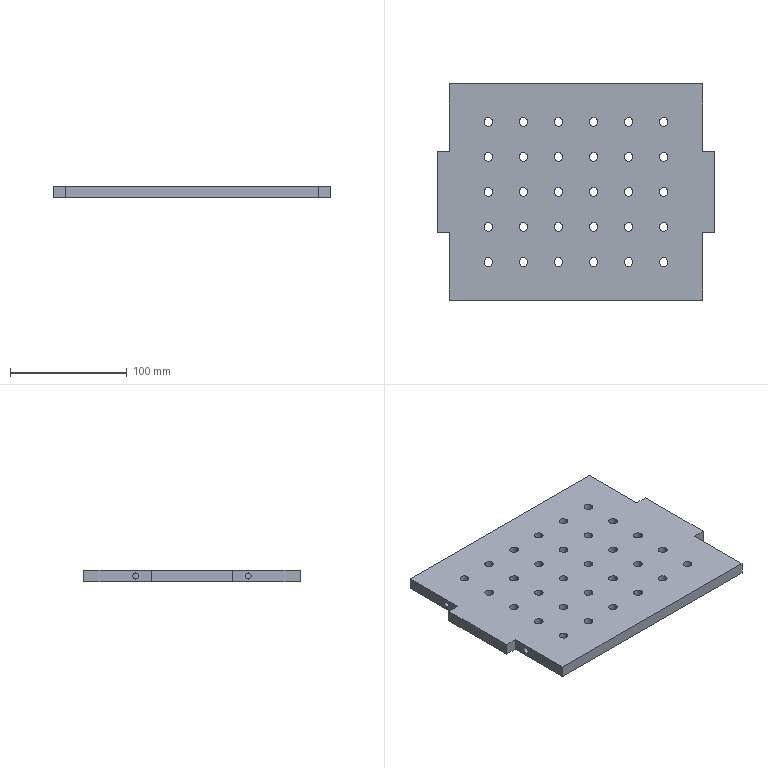CAM job | Mastercam | mm | 12 operations | part box 238 x 185 x 10
1. Contour (Ramp) | 10 - 10 平铣刀
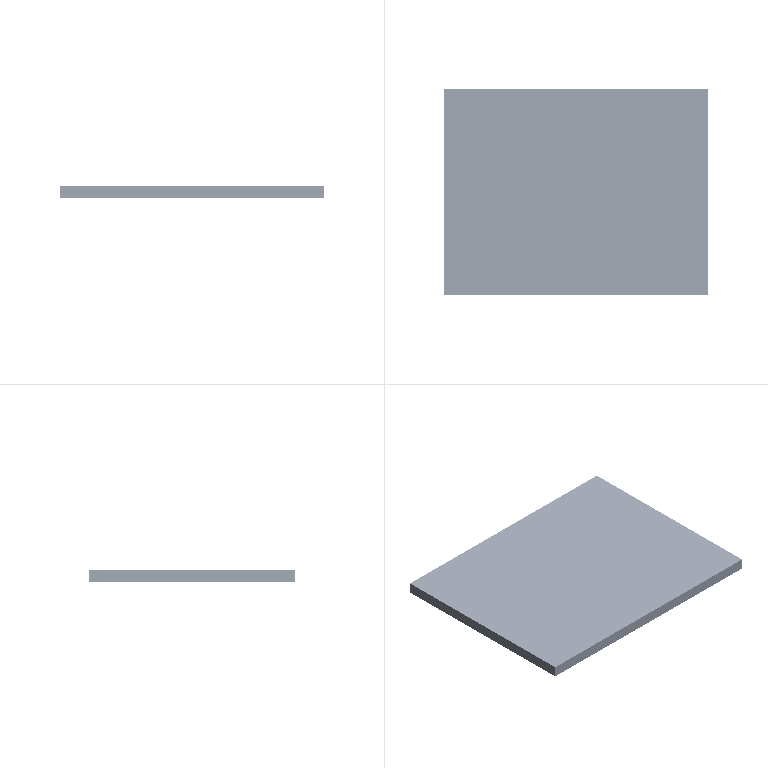2. Contour (2D) | 10 - 10 平铣刀
3. 2D High Speed (2D Area Mill) | 10 - 10 平铣刀
4. Contour (Ramp) | 10 - 10 平铣刀
5. Contour (Ramp) | 10 - 10 平铣刀
6. Contour (Ramp) | 10 - 10 平铣刀
7. Drill/Counterbore | 7 - 4 倒角刀
8. Contour (2D chamfer) | 7 - 4 倒角刀
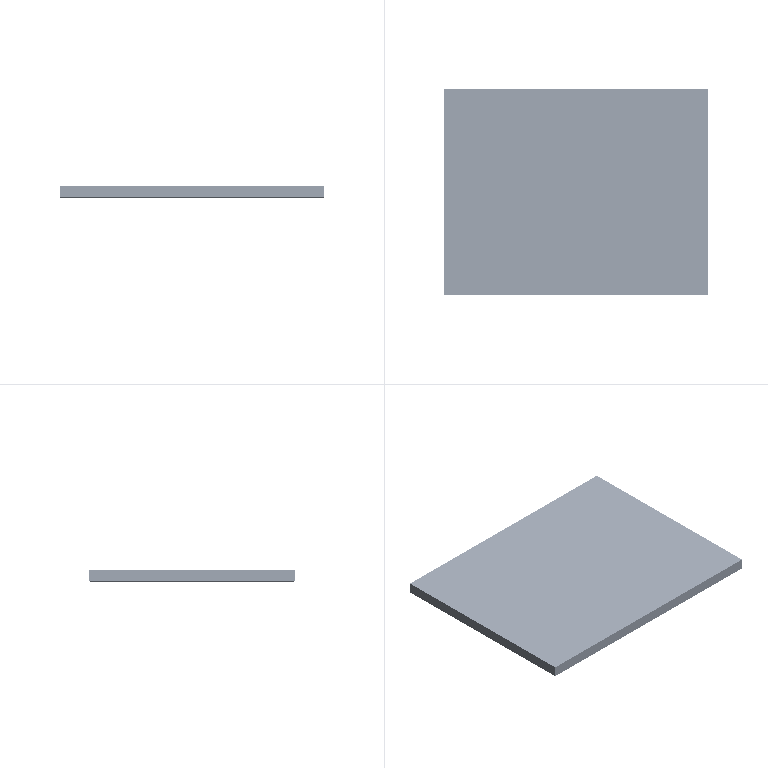9. Contour (2D) | 10 - 10 平铣刀
10. Contour (2D) | 10 - 10 平铣刀
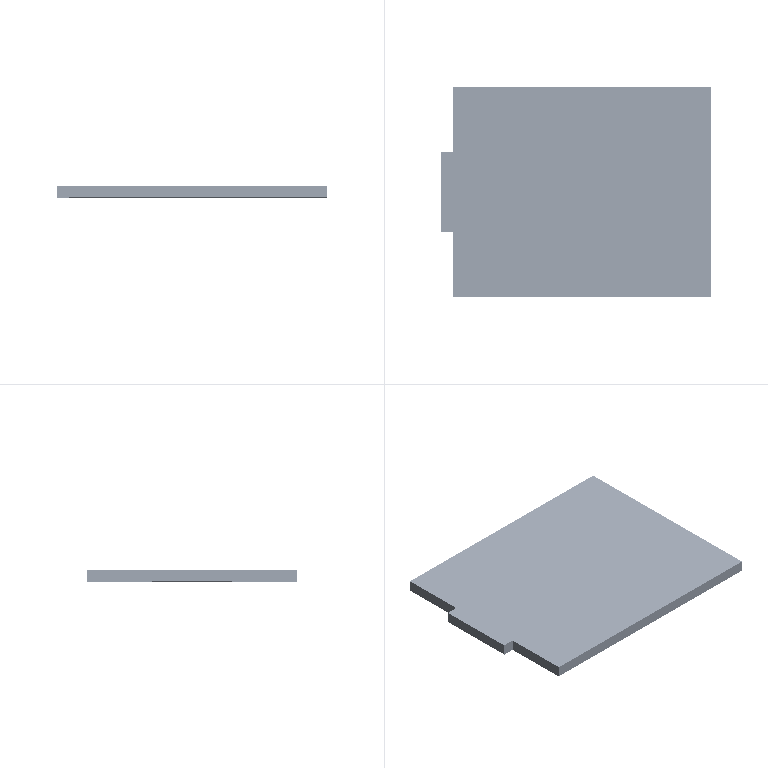11. Drill/Counterbore | 7 - 4 倒角刀
12. Model Chamfer | 7 - 4 倒角刀